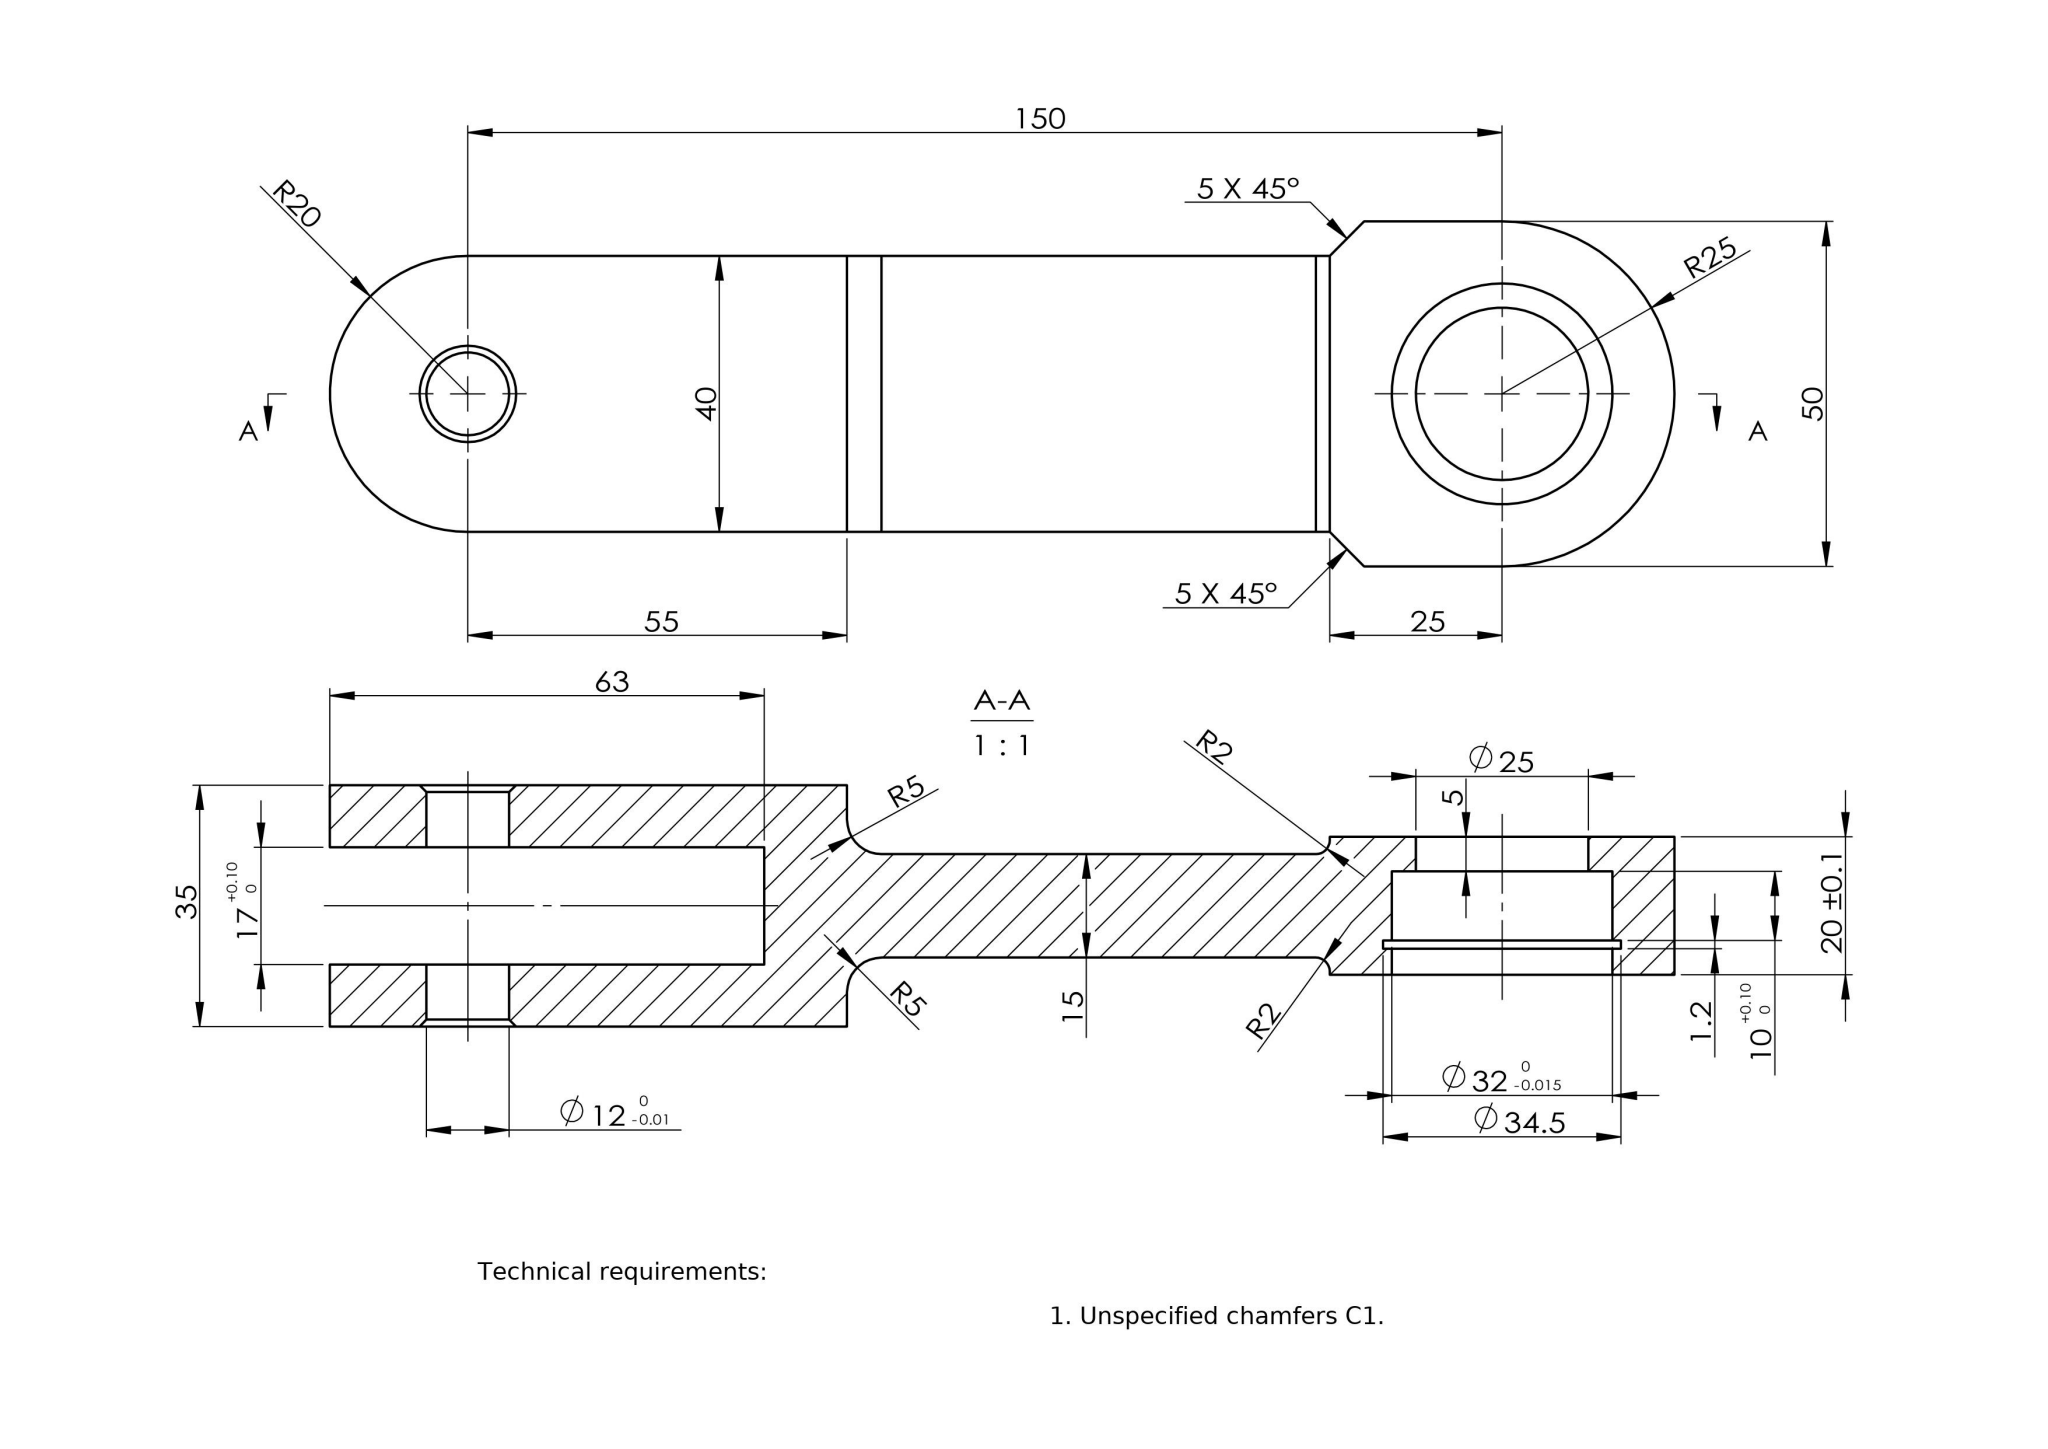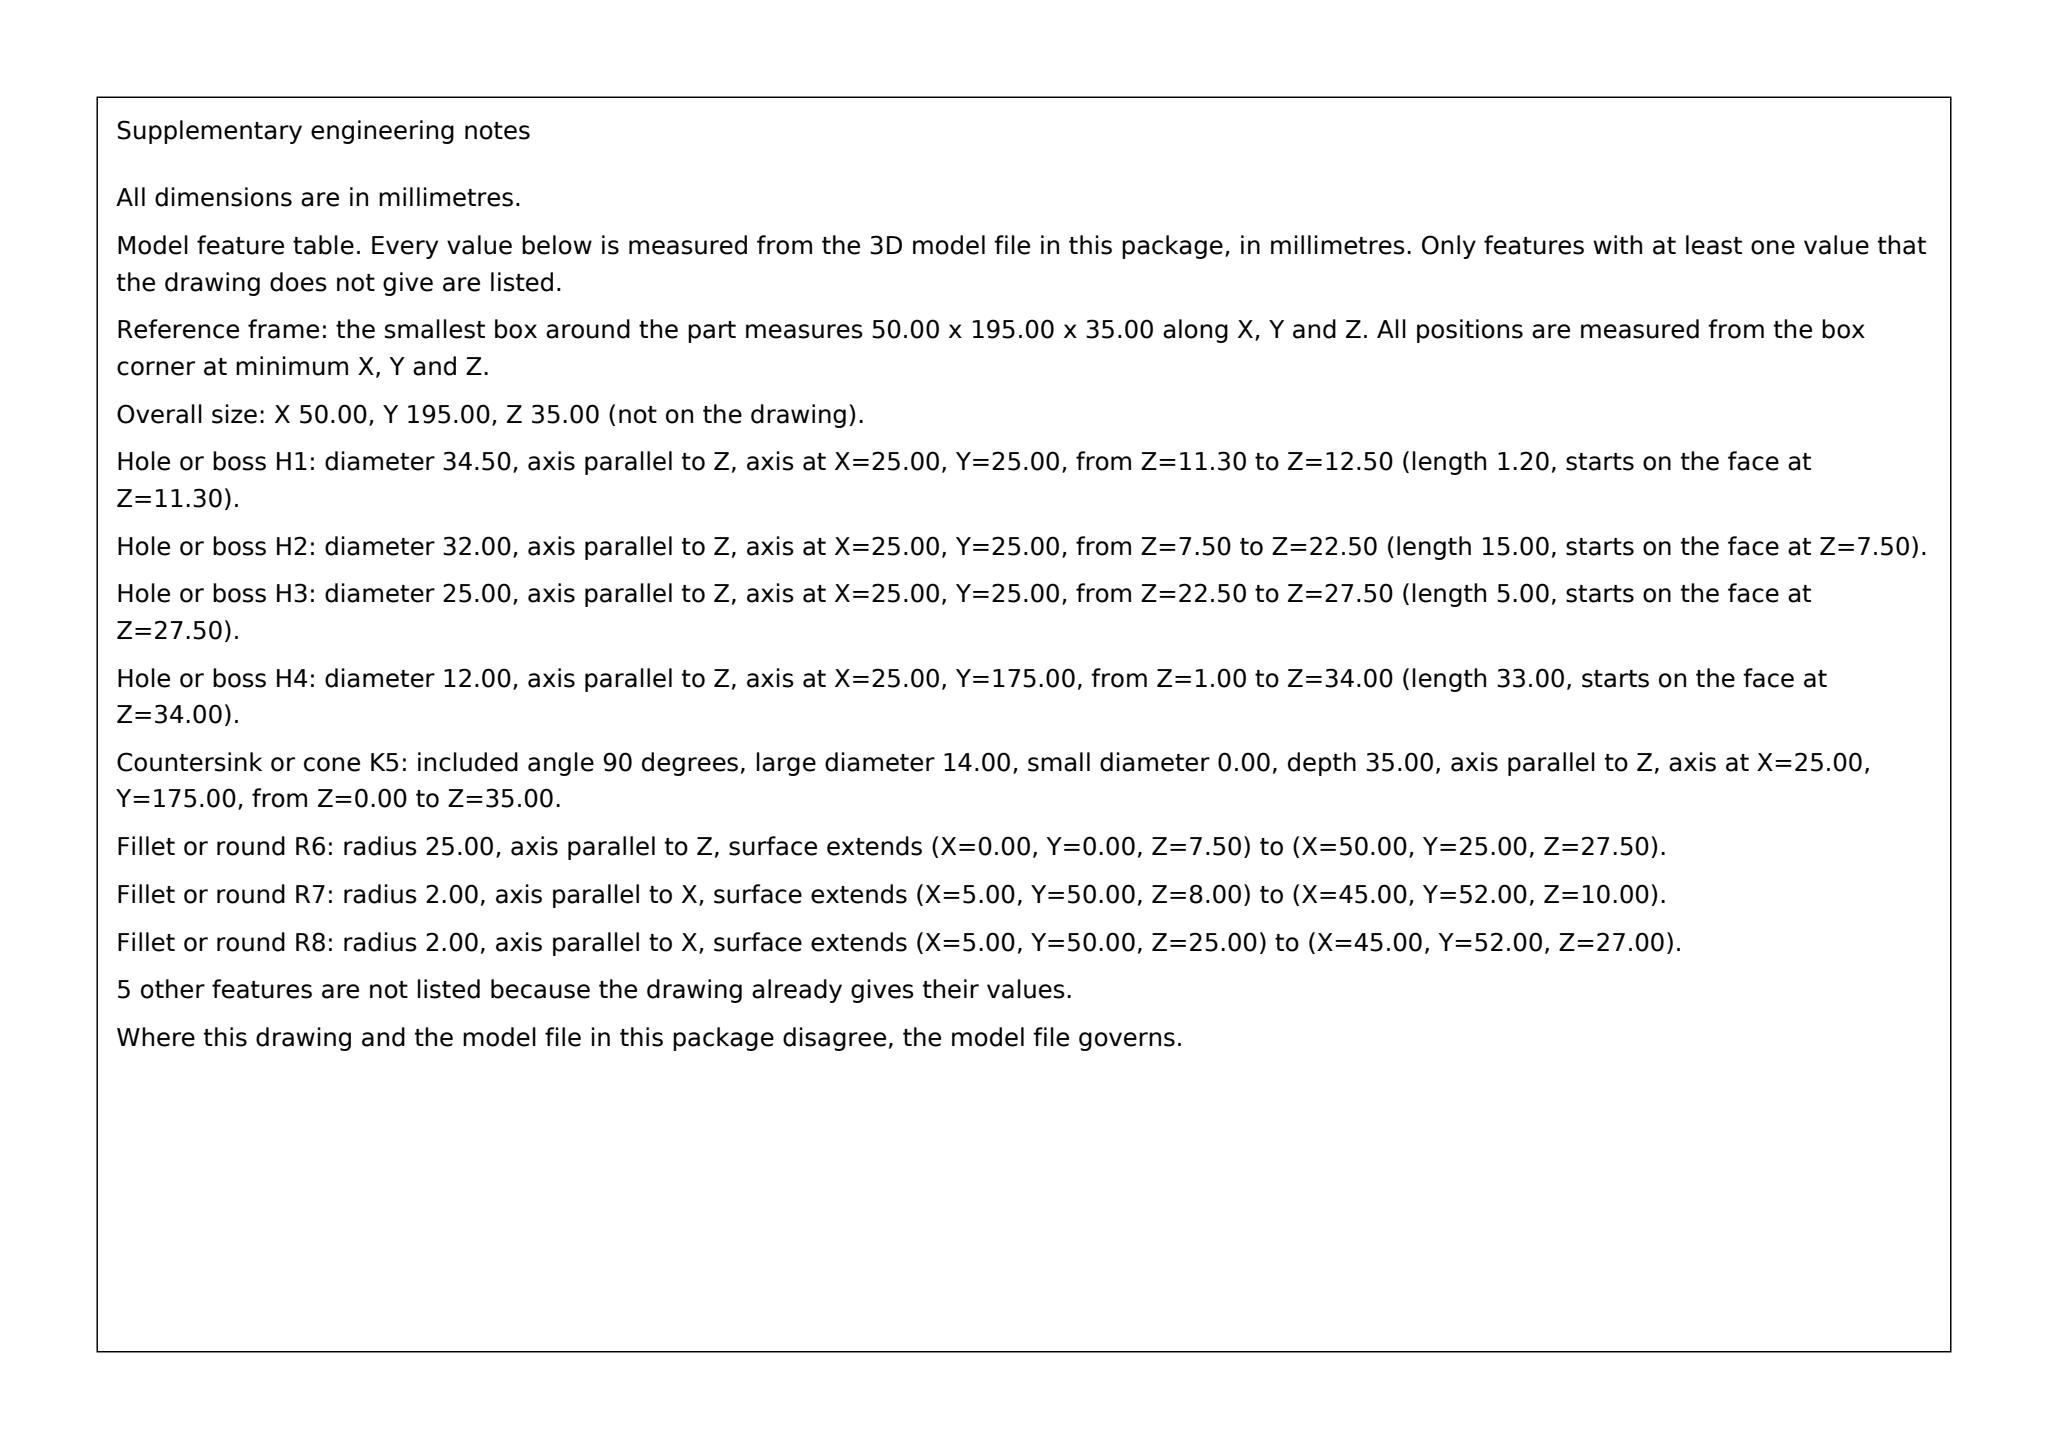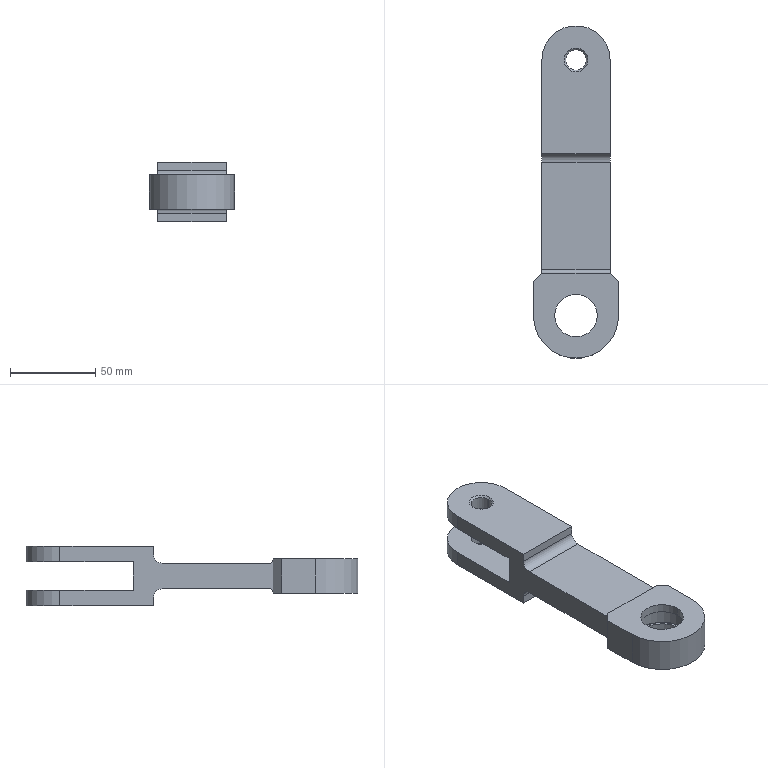Part | SolidWorks | mm | 1 solid | 45 faces | box 50 x 195 x 35 mm | volume 128952 mm3 | plane 22 | cylinder 19 | cone 4 | commonest cylinder face diameters 12 x4 32 x4 34.5 x2 25 x2 40 x2 10 x2 4 x2 50 x1